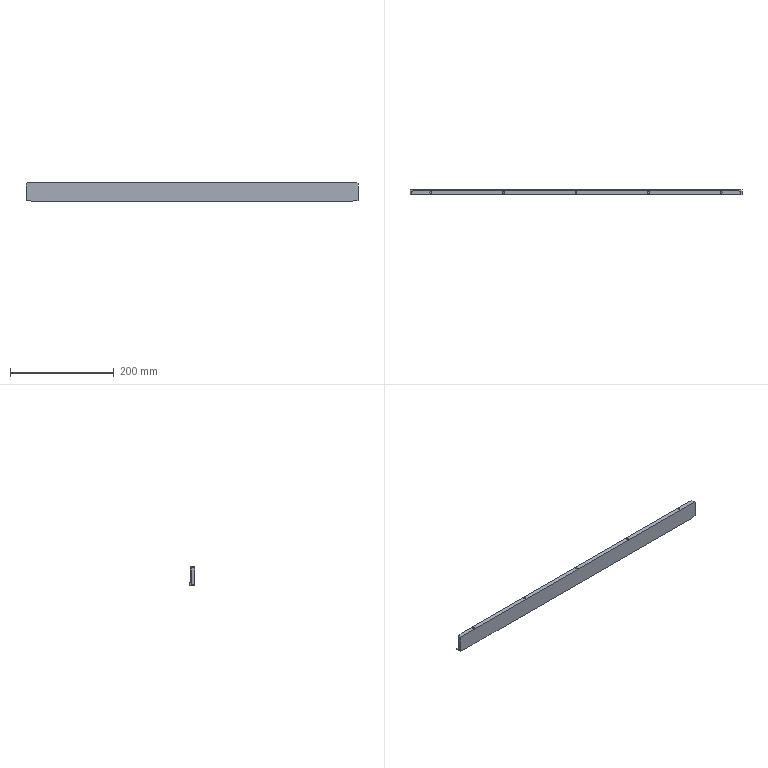Component | SolidWorks | XT-1-05-2-1 | 1 solid | 38 faces | box 640 x 10 x 35 mm | volume 184333 mm3 | plane 18 | cylinder 10 | cone 10 | commonest cylinder face diameters 3.3 x10
build123d program:
from build123d import *
from OCP.BRepFilletAPI import BRepFilletAPI_MakeChamfer

# Parameters (mm, degrees)
BOSS_EXTRUDE1_DEPTH   = 640
M4_TAPPED_HOLE1_D     = 3.3
M4_TAPPED_HOLE1_DEPTH = 10.1
M4_TAPPED_HOLE1_TIP   = 0.9914
CHAMFER1_SIZE         = 10
CHAMFER1_SIZE2        = 2
CHAMFER2_SIZE         = 1
CHAMFER2_SIZE2        = 10
CHAMFER3_SIZE         = 10
CHAMFER3_SIZE2        = 1
CHAMFER4_SIZE         = 2


with BuildPart() as part:
    # Sketch1 → Boss-Extrude1 (new body)
    with BuildSketch(Plane.XY):
        Polygon((0, 0), (0, -10), (35, -10), (35, -2), (5, -2), (5, 0), align=None)
    extrude(amount=BOSS_EXTRUDE1_DEPTH)

    # M4 Tapped Hole1
    with Locations(Plane(origin=(35, 0, 0), x_dir=(0, 0, -1), z_dir=(1, 0, 0))):
        with Locations((-600, -6), (-460, -6), (-320, -6), (-180, -6), (-40, -6)):
            Hole(M4_TAPPED_HOLE1_D / 2, depth=M4_TAPPED_HOLE1_DEPTH)
            with Locations((0, 0, -(M4_TAPPED_HOLE1_DEPTH + M4_TAPPED_HOLE1_TIP / 2))):  # 118° drill point
                Cone(0, M4_TAPPED_HOLE1_D / 2, M4_TAPPED_HOLE1_TIP, mode=Mode.SUBTRACT)

    # Chamfer1: one chamfer whose edges measure the first distance from different faces: ONE call of the kernel's chamfer builder (chamfer() names one face for all edges)
    chamfer1_edges_1 = [part.edges().sort_by_distance(p)[0] for p in [
        (20, -2, 640),
        (20, -2, 0),
    ]]
    chamfer1_side_1 = [part.faces().sort_by_distance(p)[0] for p in [
        (20, -2, 320),
    ]]
    chamfer1_edges_2 = [part.edges().sort_by_distance(p)[0] for p in [
        (5, -1, 640),
        (5, -1, 0),
    ]]
    chamfer1_side_2 = [part.faces().sort_by_distance(p)[0] for p in [
        (5, -1, 320),
    ]]
    chamfer1 = BRepFilletAPI_MakeChamfer(part.part.solid().wrapped)
    for e in chamfer1_edges_1:
        chamfer1.Add(CHAMFER1_SIZE, CHAMFER1_SIZE2, e.wrapped, chamfer1_side_1[0].wrapped)  # the first distance lies on this face
    for e in chamfer1_edges_2:
        chamfer1.Add(CHAMFER1_SIZE, CHAMFER1_SIZE2, e.wrapped, chamfer1_side_2[0].wrapped)  # the first distance lies on this face
    add(Compound.cast(chamfer1.Shape()), mode=Mode.REPLACE)

    # Chamfer2
    chamfer2_edges = [part.edges().sort_by_distance(p)[0] for p in [
        (1.5, 0, 0),
        (0, -5, 0),
    ]]
    chamfer2_side = [part.faces().sort_by_distance(p)[0] for p in [
        (16.635, -6.73, 0),
    ]]
    chamfer(chamfer2_edges, length=CHAMFER2_SIZE, length2=CHAMFER2_SIZE2, reference=chamfer2_side[0])

    # Chamfer3: one chamfer whose edges measure the first distance from different faces: ONE call of the kernel's chamfer builder (chamfer() names one face for all edges)
    chamfer3_edges_1 = [part.edges().sort_by_distance(p)[0] for p in [
        (1.5, 0, 640),
    ]]
    chamfer3_side_1 = [part.faces().sort_by_distance(p)[0] for p in [
        (2.494, 0, 324.007),
    ]]
    chamfer3_edges_2 = [part.edges().sort_by_distance(p)[0] for p in [
        (0, -5, 640),
    ]]
    chamfer3_side_2 = [part.faces().sort_by_distance(p)[0] for p in [
        (0, -5, 325),
    ]]
    chamfer3 = BRepFilletAPI_MakeChamfer(part.part.solid().wrapped)
    for e in chamfer3_edges_1:
        chamfer3.Add(CHAMFER3_SIZE, CHAMFER3_SIZE2, e.wrapped, chamfer3_side_1[0].wrapped)  # the first distance lies on this face
    for e in chamfer3_edges_2:
        chamfer3.Add(CHAMFER3_SIZE, CHAMFER3_SIZE2, e.wrapped, chamfer3_side_2[0].wrapped)  # the first distance lies on this face
    add(Compound.cast(chamfer3.Shape()), mode=Mode.REPLACE)

    # Chamfer4
    chamfer4_edges = [part.edges().sort_by_distance(p)[0] for p in [
        (35, -7, 640),
        (35, -7, 0),
    ]]
    chamfer(chamfer4_edges, length=CHAMFER4_SIZE)


solid = part.part

# Placed as in the assembly
solid = solid.moved(Location((909.283, 131.385, -42.5), (0, -90, 0)))
STEP:
#1=COLOUR_RGB('',0.7922,0.8196,0.9333);
#2=FILL_AREA_STYLE_COLOUR('',#1);
#3=FILL_AREA_STYLE('',(#2));
#4=SURFACE_STYLE_FILL_AREA(#3);
#5=SURFACE_SIDE_STYLE('',(#4));
#6=SURFACE_STYLE_USAGE(.BOTH.,#5);
#7=PRESENTATION_STYLE_ASSIGNMENT((#6));
#8=CARTESIAN_POINT('',(12.112,4.936,-0.6929));
#9=VERTEX_POINT('',#8);
#10=CARTESIAN_POINT('',(12.241,4.936,-0.6929));
#11=VERTEX_POINT('',#10);
#12=CARTESIAN_POINT('',(12.177,4.936,-0.6929));
#13=DIRECTION('',(0.,0.,1.));
#14=DIRECTION('',(1.,0.,0.));
#15=AXIS2_PLACEMENT_3D('',#12,#13,#14);
#16=CIRCLE('',#15,0.06496);
#17=EDGE_CURVE('',#9,#11,#16,.T.);
#18=ORIENTED_EDGE('',*,*,#17,.F.);
#19=CARTESIAN_POINT('',(12.112,4.936,-0.2953));
#20=VERTEX_POINT('',#19);
#21=CARTESIAN_POINT('',(12.112,4.936,-0.2953));
#22=DIRECTION('',(0.,0.,1.));
#23=VECTOR('',#22,39.37);
#24=LINE('',#21,#23);
#25=EDGE_CURVE('',#9,#20,#24,.T.);
#26=ORIENTED_EDGE('',*,*,#25,.T.);
#27=CARTESIAN_POINT('',(12.241,4.936,-0.2953));
#28=VERTEX_POINT('',#27);
#29=CARTESIAN_POINT('',(12.177,4.936,-0.2953));
#30=DIRECTION('',(0.,0.,1.));
#31=DIRECTION('',(1.,0.,0.));
#32=AXIS2_PLACEMENT_3D('',#29,#30,#31);
#33=CIRCLE('',#32,0.06496);
#34=EDGE_CURVE('',#20,#28,#33,.T.);
#35=ORIENTED_EDGE('',*,*,#34,.T.);
#36=CARTESIAN_POINT('',(12.241,4.936,-0.2953));
#37=DIRECTION('',(0.,0.,1.));
#38=VECTOR('',#37,39.37);
#39=LINE('',#36,#38);
#40=EDGE_CURVE('',#11,#28,#39,.T.);
#41=ORIENTED_EDGE('',*,*,#40,.F.);
#42=EDGE_LOOP('',(#18,#26,#35,#41));
#43=FACE_OUTER_BOUND('',#42,.T.);
#44=CARTESIAN_POINT('',(12.177,4.936,-0.2953));
#45=DIRECTION('',(0.,0.,1.));
#46=DIRECTION('',(1.,0.,0.));
#47=AXIS2_PLACEMENT_3D('',#44,#45,#46);
#48=CYLINDRICAL_SURFACE('',#47,0.06496);
#49=ADVANCED_FACE('',(#43),#48,.F.);
#50=CARTESIAN_POINT('',(12.177,4.936,-0.7319));
#51=VERTEX_POINT('',#50);
#52=CARTESIAN_POINT('',(12.241,4.936,-0.6929));
#53=DIRECTION('',(0.8572,0.,0.515));
#54=VECTOR('',#53,39.37);
#55=LINE('',#52,#54);
#56=EDGE_CURVE('',#51,#11,#55,.T.);
#57=ORIENTED_EDGE('',*,*,#56,.F.);
#58=CARTESIAN_POINT('',(12.112,4.936,-0.6929));
#59=DIRECTION('',(-0.8572,0.,0.515));
#60=VECTOR('',#59,39.37);
#61=LINE('',#58,#60);
#62=EDGE_CURVE('',#51,#9,#61,.T.);
#63=ORIENTED_EDGE('',*,*,#62,.T.);
#64=ORIENTED_EDGE('',*,*,#17,.T.);
#65=EDGE_LOOP('',(#57,#63,#64));
#66=FACE_OUTER_BOUND('',#65,.T.);
#67=CARTESIAN_POINT('',(12.177,4.936,-0.6929));
#68=DIRECTION('',(0.,0.,1.));
#69=DIRECTION('',(1.,0.,0.));
#70=AXIS2_PLACEMENT_3D('',#67,#68,#69);
#71=CONICAL_SURFACE('',#70,0.06496,1.03);
#72=ADVANCED_FACE('',(#66),#71,.F.);
#73=CARTESIAN_POINT('',(17.623,4.936,-0.6929));
#74=VERTEX_POINT('',#73);
#75=CARTESIAN_POINT('',(17.753,4.936,-0.6929));
#76=VERTEX_POINT('',#75);
#77=CARTESIAN_POINT('',(17.688,4.936,-0.6929));
#78=DIRECTION('',(0.,0.,1.));
#79=DIRECTION('',(1.,0.,0.));
#80=AXIS2_PLACEMENT_3D('',#77,#78,#79);
#81=CIRCLE('',#80,0.06496);
#82=EDGE_CURVE('',#74,#76,#81,.T.);
#83=ORIENTED_EDGE('',*,*,#82,.F.);
#84=CARTESIAN_POINT('',(17.623,4.936,-0.2953));
#85=VERTEX_POINT('',#84);
#86=CARTESIAN_POINT('',(17.623,4.936,-0.2953));
#87=DIRECTION('',(0.,0.,1.));
#88=VECTOR('',#87,39.37);
#89=LINE('',#86,#88);
#90=EDGE_CURVE('',#74,#85,#89,.T.);
#91=ORIENTED_EDGE('',*,*,#90,.T.);
#92=CARTESIAN_POINT('',(17.753,4.936,-0.2953));
#93=VERTEX_POINT('',#92);
#94=CARTESIAN_POINT('',(17.688,4.936,-0.2953));
#95=DIRECTION('',(0.,0.,1.));
#96=DIRECTION('',(1.,0.,0.));
#97=AXIS2_PLACEMENT_3D('',#94,#95,#96);
#98=CIRCLE('',#97,0.06496);
#99=EDGE_CURVE('',#85,#93,#98,.T.);
#100=ORIENTED_EDGE('',*,*,#99,.T.);
#101=CARTESIAN_POINT('',(17.753,4.936,-0.2953));
#102=DIRECTION('',(0.,0.,1.));
#103=VECTOR('',#102,39.37);
#104=LINE('',#101,#103);
#105=EDGE_CURVE('',#76,#93,#104,.T.);
#106=ORIENTED_EDGE('',*,*,#105,.F.);
#107=EDGE_LOOP('',(#83,#91,#100,#106));
#108=FACE_OUTER_BOUND('',#107,.T.);
#109=CARTESIAN_POINT('',(17.688,4.936,-0.2953));
#110=DIRECTION('',(0.,0.,1.));
#111=DIRECTION('',(1.,0.,0.));
#112=AXIS2_PLACEMENT_3D('',#109,#110,#111);
#113=CYLINDRICAL_SURFACE('',#112,0.06496);
#114=ADVANCED_FACE('',(#108),#113,.F.);
#115=CARTESIAN_POINT('',(17.688,4.936,-0.7319));
#116=VERTEX_POINT('',#115);
#117=CARTESIAN_POINT('',(17.753,4.936,-0.6929));
#118=DIRECTION('',(0.8572,0.,0.515));
#119=VECTOR('',#118,39.37);
#120=LINE('',#117,#119);
#121=EDGE_CURVE('',#116,#76,#120,.T.);
#122=ORIENTED_EDGE('',*,*,#121,.F.);
#123=CARTESIAN_POINT('',(17.623,4.936,-0.6929));
#124=DIRECTION('',(-0.8572,0.,0.515));
#125=VECTOR('',#124,39.37);
#126=LINE('',#123,#125);
#127=EDGE_CURVE('',#116,#74,#126,.T.);
#128=ORIENTED_EDGE('',*,*,#127,.T.);
#129=ORIENTED_EDGE('',*,*,#82,.T.);
#130=EDGE_LOOP('',(#122,#128,#129));
#131=FACE_OUTER_BOUND('',#130,.T.);
#132=CARTESIAN_POINT('',(17.688,4.936,-0.6929));
#133=DIRECTION('',(0.,0.,1.));
#134=DIRECTION('',(1.,0.,0.));
#135=AXIS2_PLACEMENT_3D('',#132,#133,#134);
#136=CONICAL_SURFACE('',#135,0.06496,1.03);
#137=ADVANCED_FACE('',(#131),#136,.F.);
#138=CARTESIAN_POINT('',(23.135,4.936,-0.6929));
#139=VERTEX_POINT('',#138);
#140=CARTESIAN_POINT('',(23.265,4.936,-0.6929));
#141=VERTEX_POINT('',#140);
#142=CARTESIAN_POINT('',(23.2,4.936,-0.6929));
#143=DIRECTION('',(0.,0.,1.));
#144=DIRECTION('',(1.,0.,0.));
#145=AXIS2_PLACEMENT_3D('',#142,#143,#144);
#146=CIRCLE('',#145,0.06496);
#147=EDGE_CURVE('',#139,#141,#146,.T.);
#148=ORIENTED_EDGE('',*,*,#147,.F.);
#149=CARTESIAN_POINT('',(23.135,4.936,-0.2953));
#150=VERTEX_POINT('',#149);
#151=CARTESIAN_POINT('',(23.135,4.936,-0.2953));
#152=DIRECTION('',(0.,0.,1.));
#153=VECTOR('',#152,39.37);
#154=LINE('',#151,#153);
#155=EDGE_CURVE('',#139,#150,#154,.T.);
#156=ORIENTED_EDGE('',*,*,#155,.T.);
#157=CARTESIAN_POINT('',(23.265,4.936,-0.2953));
#158=VERTEX_POINT('',#157);
#159=CARTESIAN_POINT('',(23.2,4.936,-0.2953));
#160=DIRECTION('',(0.,0.,1.));
#161=DIRECTION('',(1.,0.,0.));
#162=AXIS2_PLACEMENT_3D('',#159,#160,#161);
#163=CIRCLE('',#162,0.06496);
#164=EDGE_CURVE('',#150,#158,#163,.T.);
#165=ORIENTED_EDGE('',*,*,#164,.T.);
#166=CARTESIAN_POINT('',(23.265,4.936,-0.2953));
#167=DIRECTION('',(0.,0.,1.));
#168=VECTOR('',#167,39.37);
#169=LINE('',#166,#168);
#170=EDGE_CURVE('',#141,#158,#169,.T.);
#171=ORIENTED_EDGE('',*,*,#170,.F.);
#172=EDGE_LOOP('',(#148,#156,#165,#171));
#173=FACE_OUTER_BOUND('',#172,.T.);
#174=CARTESIAN_POINT('',(23.2,4.936,-0.2953));
#175=DIRECTION('',(0.,0.,1.));
#176=DIRECTION('',(1.,0.,0.));
#177=AXIS2_PLACEMENT_3D('',#174,#175,#176);
#178=CYLINDRICAL_SURFACE('',#177,0.06496);
#179=ADVANCED_FACE('',(#173),#178,.F.);
#180=CARTESIAN_POINT('',(23.2,4.936,-0.7319));
#181=VERTEX_POINT('',#180);
#182=CARTESIAN_POINT('',(23.265,4.936,-0.6929));
#183=DIRECTION('',(0.8572,0.,0.515));
#184=VECTOR('',#183,39.37);
#185=LINE('',#182,#184);
#186=EDGE_CURVE('',#181,#141,#185,.T.);
#187=ORIENTED_EDGE('',*,*,#186,.F.);
#188=CARTESIAN_POINT('',(23.135,4.936,-0.6929));
#189=DIRECTION('',(-0.8572,0.,0.515));
#190=VECTOR('',#189,39.37);
#191=LINE('',#188,#190);
#192=EDGE_CURVE('',#181,#139,#191,.T.);
#193=ORIENTED_EDGE('',*,*,#192,.T.);
#194=ORIENTED_EDGE('',*,*,#147,.T.);
#195=EDGE_LOOP('',(#187,#193,#194));
#196=FACE_OUTER_BOUND('',#195,.T.);
#197=CARTESIAN_POINT('',(23.2,4.936,-0.6929));
#198=DIRECTION('',(0.,0.,1.));
#199=DIRECTION('',(1.,0.,0.));
#200=AXIS2_PLACEMENT_3D('',#197,#198,#199);
#201=CONICAL_SURFACE('',#200,0.06496,1.03);
#202=ADVANCED_FACE('',(#196),#201,.F.);
#203=CARTESIAN_POINT('',(28.647,4.936,-0.6929));
#204=VERTEX_POINT('',#203);
#205=CARTESIAN_POINT('',(28.777,4.936,-0.6929));
#206=VERTEX_POINT('',#205);
#207=CARTESIAN_POINT('',(28.712,4.936,-0.6929));
#208=DIRECTION('',(0.,0.,1.));
#209=DIRECTION('',(1.,0.,0.));
#210=AXIS2_PLACEMENT_3D('',#207,#208,#209);
#211=CIRCLE('',#210,0.06496);
#212=EDGE_CURVE('',#204,#206,#211,.T.);
#213=ORIENTED_EDGE('',*,*,#212,.F.);
#214=CARTESIAN_POINT('',(28.647,4.936,-0.2953));
#215=VERTEX_POINT('',#214);
#216=CARTESIAN_POINT('',(28.647,4.936,-0.2953));
#217=DIRECTION('',(0.,0.,1.));
#218=VECTOR('',#217,39.37);
#219=LINE('',#216,#218);
#220=EDGE_CURVE('',#204,#215,#219,.T.);
#221=ORIENTED_EDGE('',*,*,#220,.T.);
#222=CARTESIAN_POINT('',(28.777,4.936,-0.2953));
#223=VERTEX_POINT('',#222);
#224=CARTESIAN_POINT('',(28.712,4.936,-0.2953));
#225=DIRECTION('',(0.,0.,1.));
#226=DIRECTION('',(1.,0.,0.));
#227=AXIS2_PLACEMENT_3D('',#224,#225,#226);
#228=CIRCLE('',#227,0.06496);
#229=EDGE_CURVE('',#215,#223,#228,.T.);
#230=ORIENTED_EDGE('',*,*,#229,.T.);
#231=CARTESIAN_POINT('',(28.777,4.936,-0.2953));
#232=DIRECTION('',(0.,0.,1.));
#233=VECTOR('',#232,39.37);
#234=LINE('',#231,#233);
#235=EDGE_CURVE('',#206,#223,#234,.T.);
#236=ORIENTED_EDGE('',*,*,#235,.F.);
#237=EDGE_LOOP('',(#213,#221,#230,#236));
#238=FACE_OUTER_BOUND('',#237,.T.);
#239=CARTESIAN_POINT('',(28.712,4.936,-0.2953));
#240=DIRECTION('',(0.,0.,1.));
#241=DIRECTION('',(1.,0.,0.));
#242=AXIS2_PLACEMENT_3D('',#239,#240,#241);
#243=CYLINDRICAL_SURFACE('',#242,0.06496);
#244=ADVANCED_FACE('',(#238),#243,.F.);
#245=CARTESIAN_POINT('',(28.712,4.936,-0.7319));
#246=VERTEX_POINT('',#245);
#247=CARTESIAN_POINT('',(28.777,4.936,-0.6929));
#248=DIRECTION('',(0.8572,0.,0.515));
#249=VECTOR('',#248,39.37);
#250=LINE('',#247,#249);
#251=EDGE_CURVE('',#246,#206,#250,.T.);
#252=ORIENTED_EDGE('',*,*,#251,.F.);
#253=CARTESIAN_POINT('',(28.647,4.936,-0.6929));
#254=DIRECTION('',(-0.8572,0.,0.515));
#255=VECTOR('',#254,39.37);
#256=LINE('',#253,#255);
#257=EDGE_CURVE('',#246,#204,#256,.T.);
#258=ORIENTED_EDGE('',*,*,#257,.T.);
#259=ORIENTED_EDGE('',*,*,#212,.T.);
#260=EDGE_LOOP('',(#252,#258,#259));
#261=FACE_OUTER_BOUND('',#260,.T.);
#262=CARTESIAN_POINT('',(28.712,4.936,-0.6929));
#263=DIRECTION('',(0.,0.,1.));
#264=DIRECTION('',(1.,0.,0.));
#265=AXIS2_PLACEMENT_3D('',#262,#263,#264);
#266=CONICAL_SURFACE('',#265,0.06496,1.03);
#267=ADVANCED_FACE('',(#261),#266,.F.);
#268=CARTESIAN_POINT('',(34.159,4.936,-0.6929));
#269=VERTEX_POINT('',#268);
#270=CARTESIAN_POINT('',(34.289,4.936,-0.6929));
#271=VERTEX_POINT('',#270);
#272=CARTESIAN_POINT('',(34.224,4.936,-0.6929));
#273=DIRECTION('',(0.,0.,1.));
#274=DIRECTION('',(1.,0.,0.));
#275=AXIS2_PLACEMENT_3D('',#272,#273,#274);
#276=CIRCLE('',#275,0.06496);
#277=EDGE_CURVE('',#269,#271,#276,.T.);
#278=ORIENTED_EDGE('',*,*,#277,.F.);
#279=CARTESIAN_POINT('',(34.159,4.936,-0.2953));
#280=VERTEX_POINT('',#279);
#281=CARTESIAN_POINT('',(34.159,4.936,-0.2953));
#282=DIRECTION('',(0.,0.,1.));
#283=VECTOR('',#282,39.37);
#284=LINE('',#281,#283);
#285=EDGE_CURVE('',#269,#280,#284,.T.);
#286=ORIENTED_EDGE('',*,*,#285,.T.);
#287=CARTESIAN_POINT('',(34.289,4.936,-0.2953));
#288=VERTEX_POINT('',#287);
#289=CARTESIAN_POINT('',(34.224,4.936,-0.2953));
#290=DIRECTION('',(0.,0.,1.));
#291=DIRECTION('',(1.,0.,0.));
#292=AXIS2_PLACEMENT_3D('',#289,#290,#291);
#293=CIRCLE('',#292,0.06496);
#294=EDGE_CURVE('',#280,#288,#293,.T.);
#295=ORIENTED_EDGE('',*,*,#294,.T.);
#296=CARTESIAN_POINT('',(34.289,4.936,-0.2953));
#297=DIRECTION('',(0.,0.,1.));
#298=VECTOR('',#297,39.37);
#299=LINE('',#296,#298);
#300=EDGE_CURVE('',#271,#288,#299,.T.);
#301=ORIENTED_EDGE('',*,*,#300,.F.);
#302=EDGE_LOOP('',(#278,#286,#295,#301));
#303=FACE_OUTER_BOUND('',#302,.T.);
#304=CARTESIAN_POINT('',(34.224,4.936,-0.2953));
#305=DIRECTION('',(0.,0.,1.));
#306=DIRECTION('',(1.,0.,0.));
#307=AXIS2_PLACEMENT_3D('',#304,#305,#306);
#308=CYLINDRICAL_SURFACE('',#307,0.06496);
#309=ADVANCED_FACE('',(#303),#308,.F.);
#310=CARTESIAN_POINT('',(34.224,4.936,-0.7319));
#311=VERTEX_POINT('',#310);
#312=CARTESIAN_POINT('',(34.289,4.936,-0.6929));
#313=DIRECTION('',(0.8572,0.,0.515));
#314=VECTOR('',#313,39.37);
#315=LINE('',#312,#314);
#316=EDGE_CURVE('',#311,#271,#315,.T.);
#317=ORIENTED_EDGE('',*,*,#316,.F.);
#318=CARTESIAN_POINT('',(34.159,4.936,-0.6929));
#319=DIRECTION('',(-0.8572,0.,0.515));
#320=VECTOR('',#319,39.37);
#321=LINE('',#318,#320);
#322=EDGE_CURVE('',#311,#269,#321,.T.);
#323=ORIENTED_EDGE('',*,*,#322,.T.);
#324=ORIENTED_EDGE('',*,*,#277,.T.);
#325=EDGE_LOOP('',(#317,#323,#324));
#326=FACE_OUTER_BOUND('',#325,.T.);
#327=CARTESIAN_POINT('',(34.224,4.936,-0.6929));
#328=DIRECTION('',(0.,0.,1.));
#329=DIRECTION('',(1.,0.,0.));
#330=AXIS2_PLACEMENT_3D('',#327,#328,#329);
#331=CONICAL_SURFACE('',#330,0.06496,1.03);
#332=ADVANCED_FACE('',(#326),#331,.F.);
#333=CARTESIAN_POINT('',(10.995,5.173,-1.673));
#334=VERTEX_POINT('',#333);
#335=CARTESIAN_POINT('',(35.405,5.173,-1.673));
#336=VERTEX_POINT('',#335);
#337=CARTESIAN_POINT('',(10.602,5.173,-1.673));
#338=DIRECTION('',(1.,0.,0.));
#339=VECTOR('',#338,39.37);
#340=LINE('',#337,#339);
#341=EDGE_CURVE('',#334,#336,#340,.T.);
#342=ORIENTED_EDGE('',*,*,#341,.F.);
#343=CARTESIAN_POINT('',(10.995,5.173,-1.476));
#344=VERTEX_POINT('',#343);
#345=CARTESIAN_POINT('',(10.995,5.173,-1.555));
#346=DIRECTION('',(0.,0.,1.));
#347=VECTOR('',#346,39.37);
#348=LINE('',#345,#347);
#349=EDGE_CURVE('',#334,#344,#348,.T.);
#350=ORIENTED_EDGE('',*,*,#349,.T.);
#351=CARTESIAN_POINT('',(35.405,5.173,-1.476));
#352=VERTEX_POINT('',#351);
#353=CARTESIAN_POINT('',(10.602,5.173,-1.476));
#354=DIRECTION('',(1.,0.,0.));
#355=VECTOR('',#354,39.37);
#356=LINE('',#353,#355);
#357=EDGE_CURVE('',#344,#352,#356,.T.);
#358=ORIENTED_EDGE('',*,*,#357,.T.);
#359=CARTESIAN_POINT('',(35.405,5.173,-1.476));
#360=DIRECTION('',(0.,-0.,-1.));
#361=VECTOR('',#360,39.37);
#362=LINE('',#359,#361);
#363=EDGE_CURVE('',#352,#336,#362,.T.);
#364=ORIENTED_EDGE('',*,*,#363,.T.);
#365=EDGE_LOOP('',(#342,#350,#358,#364));
#366=FACE_OUTER_BOUND('',#365,.T.);
#367=CARTESIAN_POINT('',(10.602,5.173,-1.476));
#368=DIRECTION('',(0.,-1.,0.));
#369=DIRECTION('',(0.,0.,1.));
#370=AXIS2_PLACEMENT_3D('',#367,#368,#369);
#371=PLANE('',#370);
#372=ADVANCED_FACE('',(#366),#371,.F.);
#373=CARTESIAN_POINT('',(10.995,4.779,-1.673));
#374=VERTEX_POINT('',#373);
#375=CARTESIAN_POINT('',(35.405,4.779,-1.673));
#376=VERTEX_POINT('',#375);
#377=CARTESIAN_POINT('',(10.602,4.779,-1.673));
#378=DIRECTION('',(1.,0.,0.));
#379=VECTOR('',#378,39.37);
#380=LINE('',#377,#379);
#381=EDGE_CURVE('',#374,#376,#380,.T.);
#382=ORIENTED_EDGE('',*,*,#381,.F.);
#383=CARTESIAN_POINT('',(10.995,5.173,-1.673));
#384=DIRECTION('',(0.,1.,-0.));
#385=VECTOR('',#384,39.37);
#386=LINE('',#383,#385);
#387=EDGE_CURVE('',#374,#334,#386,.T.);
#388=ORIENTED_EDGE('',*,*,#387,.T.);
#389=ORIENTED_EDGE('',*,*,#341,.T.);
#390=CARTESIAN_POINT('',(35.405,5.173,-1.673));
#391=DIRECTION('',(0.,-1.,0.));
#392=VECTOR('',#391,39.37);
#393=LINE('',#390,#392);
#394=EDGE_CURVE('',#336,#376,#393,.T.);
#395=ORIENTED_EDGE('',*,*,#394,.T.);
#396=EDGE_LOOP('',(#382,#388,#389,#395));
#397=FACE_OUTER_BOUND('',#396,.T.);
#398=CARTESIAN_POINT('',(10.602,5.173,-1.673));
#399=DIRECTION('',(0.,0.,1.));
#400=DIRECTION('',(0.,1.,-0.));
#401=AXIS2_PLACEMENT_3D('',#398,#399,#400);
#402=PLANE('',#401);
#403=ADVANCED_FACE('',(#397),#402,.F.);
#404=CARTESIAN_POINT('',(35.799,4.779,-1.634));
#405=VERTEX_POINT('',#404);
#406=CARTESIAN_POINT('',(35.799,4.779,-0.374));
#407=VERTEX_POINT('',#406);
#408=CARTESIAN_POINT('',(35.799,4.779,-1.673));
#409=DIRECTION('',(0.,0.,1.));
#410=VECTOR('',#409,39.37);
#411=LINE('',#408,#410);
#412=EDGE_CURVE('',#405,#407,#411,.T.);
#413=ORIENTED_EDGE('',*,*,#412,.T.);
#414=CARTESIAN_POINT('',(35.72,4.779,-0.2953));
#415=VERTEX_POINT('',#414);
#416=CARTESIAN_POINT('',(35.72,4.779,-0.2953));
#417=DIRECTION('',(-0.7071,0.,0.7071));
#418=VECTOR('',#417,39.37);
#419=LINE('',#416,#418);
#420=EDGE_CURVE('',#407,#415,#419,.T.);
#421=ORIENTED_EDGE('',*,*,#420,.T.);
#422=CARTESIAN_POINT('',(10.68,4.779,-0.2953));
#423=VERTEX_POINT('',#422);
#424=CARTESIAN_POINT('',(10.602,4.779,-0.2953));
#425=DIRECTION('',(1.,0.,0.));
#426=VECTOR('',#425,39.37);
#427=LINE('',#424,#426);
#428=EDGE_CURVE('',#423,#415,#427,.T.);
#429=ORIENTED_EDGE('',*,*,#428,.F.);
#430=CARTESIAN_POINT('',(10.602,4.779,-0.374));
#431=VERTEX_POINT('',#430);
#432=CARTESIAN_POINT('',(10.602,4.779,-0.374));
#433=DIRECTION('',(-0.7071,-0.,-0.7071));
#434=VECTOR('',#433,39.37);
#435=LINE('',#432,#434);
#436=EDGE_CURVE('',#423,#431,#435,.T.);
#437=ORIENTED_EDGE('',*,*,#436,.T.);
#438=CARTESIAN_POINT('',(10.602,4.779,-1.634));
#439=VERTEX_POINT('',#438);
#440=CARTESIAN_POINT('',(10.602,4.779,-1.673));
#441=DIRECTION('',(0.,0.,1.));
#442=VECTOR('',#441,39.37);
#443=LINE('',#440,#442);
#444=EDGE_CURVE('',#439,#431,#443,.T.);
#445=ORIENTED_EDGE('',*,*,#444,.F.);
#446=CARTESIAN_POINT('',(10.602,4.779,-1.634));
#447=DIRECTION('',(0.995,-0.,-0.0995));
#448=VECTOR('',#447,39.37);
#449=LINE('',#446,#448);
#450=EDGE_CURVE('',#439,#374,#449,.T.);
#451=ORIENTED_EDGE('',*,*,#450,.T.);
#452=ORIENTED_EDGE('',*,*,#381,.T.);
#453=CARTESIAN_POINT('',(35.405,4.779,-1.673));
#454=DIRECTION('',(0.995,0.,0.0995));
#455=VECTOR('',#454,39.37);
#456=LINE('',#453,#455);
#457=EDGE_CURVE('',#376,#405,#456,.T.);
#458=ORIENTED_EDGE('',*,*,#457,.T.);
#459=EDGE_LOOP('',(#413,#421,#429,#437,#445,#451,#452,#458));
#460=FACE_OUTER_BOUND('',#459,.T.);
#461=CARTESIAN_POINT('',(10.602,4.779,-1.673));
#462=DIRECTION('',(0.,1.,-0.));
#463=DIRECTION('',(0.,-0.,-1.));
#464=AXIS2_PLACEMENT_3D('',#461,#462,#463);
#465=PLANE('',#464);
#466=ADVANCED_FACE('',(#460),#465,.F.);
#467=CARTESIAN_POINT('',(12.177,4.936,-0.2953));
#468=DIRECTION('',(0.,0.,1.));
#469=DIRECTION('',(1.,0.,0.));
#470=AXIS2_PLACEMENT_3D('',#467,#468,#469);
#471=CIRCLE('',#470,0.06496);
#472=EDGE_CURVE('',#28,#20,#471,.T.);
#473=ORIENTED_EDGE('',*,*,#472,.F.);
#474=ORIENTED_EDGE('',*,*,#34,.F.);
#475=EDGE_LOOP('',(#473,#474));
#476=FACE_BOUND('',#475,.T.);
#477=CARTESIAN_POINT('',(17.688,4.936,-0.2953));
#478=DIRECTION('',(0.,0.,1.));
#479=DIRECTION('',(1.,0.,0.));
#480=AXIS2_PLACEMENT_3D('',#477,#478,#479);
#481=CIRCLE('',#480,0.06496);
#482=EDGE_CURVE('',#93,#85,#481,.T.);
#483=ORIENTED_EDGE('',*,*,#482,.F.);
#484=ORIENTED_EDGE('',*,*,#99,.F.);
#485=EDGE_LOOP('',(#483,#484));
#486=FACE_BOUND('',#485,.T.);
#487=CARTESIAN_POINT('',(23.2,4.936,-0.2953));
#488=DIRECTION('',(0.,0.,1.));
#489=DIRECTION('',(1.,0.,0.));
#490=AXIS2_PLACEMENT_3D('',#487,#488,#489);
#491=CIRCLE('',#490,0.06496);
#492=EDGE_CURVE('',#158,#150,#491,.T.);
#493=ORIENTED_EDGE('',*,*,#492,.F.);
#494=ORIENTED_EDGE('',*,*,#164,.F.);
#495=EDGE_LOOP('',(#493,#494));
#496=FACE_BOUND('',#495,.T.);
#497=CARTESIAN_POINT('',(28.712,4.936,-0.2953));
#498=DIRECTION('',(0.,0.,1.));
#499=DIRECTION('',(1.,0.,0.));
#500=AXIS2_PLACEMENT_3D('',#497,#498,#499);
#501=CIRCLE('',#500,0.06496);
#502=EDGE_CURVE('',#223,#215,#501,.T.);
#503=ORIENTED_EDGE('',*,*,#502,.F.);
#504=ORIENTED_EDGE('',*,*,#229,.F.);
#505=EDGE_LOOP('',(#503,#504));
#506=FACE_BOUND('',#505,.T.);
#507=CARTESIAN_POINT('',(34.224,4.936,-0.2953));
#508=DIRECTION('',(0.,0.,1.));
#509=DIRECTION('',(1.,0.,0.));
#510=AXIS2_PLACEMENT_3D('',#507,#508,#509);
#511=CIRCLE('',#510,0.06496);
#512=EDGE_CURVE('',#288,#280,#511,.T.);
#513=ORIENTED_EDGE('',*,*,#512,.F.);
#514=ORIENTED_EDGE('',*,*,#294,.F.);
#515=EDGE_LOOP('',(#513,#514));
#516=FACE_BOUND('',#515,.T.);
#517=ORIENTED_EDGE('',*,*,#428,.T.);
#518=CARTESIAN_POINT('',(35.72,5.031,-0.2953));
#519=VERTEX_POINT('',#518);
#520=CARTESIAN_POINT('',(35.72,4.779,-0.2953));
#521=DIRECTION('',(0.,1.,0.));
#522=VECTOR('',#521,39.37);
#523=LINE('',#520,#522);
#524=EDGE_CURVE('',#415,#519,#523,.T.);
#525=ORIENTED_EDGE('',*,*,#524,.T.);
#526=CARTESIAN_POINT('',(35.405,5.094,-0.2953));
#527=VERTEX_POINT('',#526);
#528=CARTESIAN_POINT('',(35.405,5.094,-0.2953));
#529=DIRECTION('',(-0.9806,0.1961,0.));
#530=VECTOR('',#529,39.37);
#531=LINE('',#528,#530);
#532=EDGE_CURVE('',#519,#527,#531,.T.);
#533=ORIENTED_EDGE('',*,*,#532,.T.);
#534=CARTESIAN_POINT('',(10.995,5.094,-0.2953));
#535=VERTEX_POINT('',#534);
#536=CARTESIAN_POINT('',(10.602,5.094,-0.2953));
#537=DIRECTION('',(1.,0.,0.));
#538=VECTOR('',#537,39.37);
#539=LINE('',#536,#538);
#540=EDGE_CURVE('',#535,#527,#539,.T.);
#541=ORIENTED_EDGE('',*,*,#540,.F.);
#542=CARTESIAN_POINT('',(10.68,5.031,-0.2953));
#543=VERTEX_POINT('',#542);
#544=CARTESIAN_POINT('',(10.602,5.015,-0.2953));
#545=DIRECTION('',(-0.9806,-0.1961,0.));
#546=VECTOR('',#545,39.37);
#547=LINE('',#544,#546);
#548=EDGE_CURVE('',#535,#543,#547,.T.);
#549=ORIENTED_EDGE('',*,*,#548,.T.);
#550=CARTESIAN_POINT('',(10.68,4.779,-0.2953));
#551=DIRECTION('',(0.,-1.,0.));
#552=VECTOR('',#551,39.37);
#553=LINE('',#550,#552);
#554=EDGE_CURVE('',#543,#423,#553,.T.);
#555=ORIENTED_EDGE('',*,*,#554,.T.);
#556=EDGE_LOOP('',(#517,#525,#533,#541,#549,#555));
#557=FACE_OUTER_BOUND('',#556,.T.);
#558=CARTESIAN_POINT('',(10.602,4.779,-0.2953));
#559=DIRECTION('',(0.,0.,-1.));
#560=DIRECTION('',(-1.,0.,0.));
#561=AXIS2_PLACEMENT_3D('',#558,#559,#560);
#562=PLANE('',#561);
#563=ADVANCED_FACE('',(#476,#486,#496,#506,#516,#557),#562,.F.);
#564=ORIENTED_EDGE('',*,*,#540,.T.);
#565=CARTESIAN_POINT('',(35.405,5.094,-1.476));
#566=VERTEX_POINT('',#565);
#567=CARTESIAN_POINT('',(35.405,5.094,-0.2953));
#568=DIRECTION('',(0.,-0.,-1.));
#569=VECTOR('',#568,39.37);
#570=LINE('',#567,#569);
#571=EDGE_CURVE('',#527,#566,#570,.T.);
#572=ORIENTED_EDGE('',*,*,#571,.T.);
#573=CARTESIAN_POINT('',(10.995,5.094,-1.476));
#574=VERTEX_POINT('',#573);
#575=CARTESIAN_POINT('',(10.602,5.094,-1.476));
#576=DIRECTION('',(1.,0.,0.));
#577=VECTOR('',#576,39.37);
#578=LINE('',#575,#577);
#579=EDGE_CURVE('',#574,#566,#578,.T.);
#580=ORIENTED_EDGE('',*,*,#579,.F.);
#581=CARTESIAN_POINT('',(10.995,5.094,-0.2953));
#582=DIRECTION('',(0.,0.,1.));
#583=VECTOR('',#582,39.37);
#584=LINE('',#581,#583);
#585=EDGE_CURVE('',#574,#535,#584,.T.);
#586=ORIENTED_EDGE('',*,*,#585,.T.);
#587=EDGE_LOOP('',(#564,#572,#580,#586));
#588=FACE_OUTER_BOUND('',#587,.T.);
#589=CARTESIAN_POINT('',(10.602,5.094,-0.2953));
#590=DIRECTION('',(0.,-1.,0.));
#591=DIRECTION('',(0.,0.,1.));
#592=AXIS2_PLACEMENT_3D('',#589,#590,#591);
#593=PLANE('',#592);
#594=ADVANCED_FACE('',(#588),#593,.F.);
#595=ORIENTED_EDGE('',*,*,#579,.T.);
#596=CARTESIAN_POINT('',(35.405,5.094,-1.476));
#597=DIRECTION('',(0.,1.,0.));
#598=VECTOR('',#597,39.37);
#599=LINE('',#596,#598);
#600=EDGE_CURVE('',#566,#352,#599,.T.);
#601=ORIENTED_EDGE('',*,*,#600,.T.);
#602=ORIENTED_EDGE('',*,*,#357,.F.);
#603=CARTESIAN_POINT('',(10.995,5.094,-1.476));
#604=DIRECTION('',(0.,-1.,0.));
#605=VECTOR('',#604,39.37);
#606=LINE('',#603,#605);
#607=EDGE_CURVE('',#344,#574,#606,.T.);
#608=ORIENTED_EDGE('',*,*,#607,.T.);
#609=EDGE_LOOP('',(#595,#601,#602,#608));
#610=FACE_OUTER_BOUND('',#609,.T.);
#611=CARTESIAN_POINT('',(10.602,5.094,-1.476));
#612=DIRECTION('',(0.,0.,-1.));
#613=DIRECTION('',(-1.,0.,0.));
#614=AXIS2_PLACEMENT_3D('',#611,#612,#613);
#615=PLANE('',#614);
#616=ADVANCED_FACE('',(#610),#615,.F.);
#617=ORIENTED_EDGE('',*,*,#444,.T.);
#618=CARTESIAN_POINT('',(10.602,5.015,-0.374));
#619=VERTEX_POINT('',#618);
#620=CARTESIAN_POINT('',(10.602,5.015,-0.374));
#621=DIRECTION('',(0.,1.,0.));
#622=VECTOR('',#621,39.37);
#623=LINE('',#620,#622);
#624=EDGE_CURVE('',#431,#619,#623,.T.);
#625=ORIENTED_EDGE('',*,*,#624,.T.);
#626=CARTESIAN_POINT('',(10.602,5.015,-1.555));
#627=VERTEX_POINT('',#626);
#628=CARTESIAN_POINT('',(10.602,5.015,-1.476));
#629=DIRECTION('',(0.,-0.,-1.));
#630=VECTOR('',#629,39.37);
#631=LINE('',#628,#630);
#632=EDGE_CURVE('',#619,#627,#631,.T.);
#633=ORIENTED_EDGE('',*,*,#632,.T.);
#634=CARTESIAN_POINT('',(10.602,5.133,-1.555));
#635=VERTEX_POINT('',#634);
#636=CARTESIAN_POINT('',(10.602,5.173,-1.555));
#637=DIRECTION('',(0.,1.,0.));
#638=VECTOR('',#637,39.37);
#639=LINE('',#636,#638);
#640=EDGE_CURVE('',#627,#635,#639,.T.);
#641=ORIENTED_EDGE('',*,*,#640,.T.);
#642=CARTESIAN_POINT('',(10.602,5.133,-1.634));
#643=VERTEX_POINT('',#642);
#644=CARTESIAN_POINT('',(10.602,5.133,-1.673));
#645=DIRECTION('',(0.,-0.,-1.));
#646=VECTOR('',#645,39.37);
#647=LINE('',#644,#646);
#648=EDGE_CURVE('',#635,#643,#647,.T.);
#649=ORIENTED_EDGE('',*,*,#648,.T.);
#650=CARTESIAN_POINT('',(10.602,4.779,-1.634));
#651=DIRECTION('',(0.,-1.,0.));
#652=VECTOR('',#651,39.37);
#653=LINE('',#650,#652);
#654=EDGE_CURVE('',#643,#439,#653,.T.);
#655=ORIENTED_EDGE('',*,*,#654,.T.);
#656=EDGE_LOOP('',(#617,#625,#633,#641,#649,#655));
#657=FACE_OUTER_BOUND('',#656,.T.);
#658=CARTESIAN_POINT('',(10.602,5.173,-1.673));
#659=DIRECTION('',(-1.,0.,0.));
#660=DIRECTION('',(0.,0.,1.));
#661=AXIS2_PLACEMENT_3D('',#658,#659,#660);
#662=PLANE('',#661);
#663=ADVANCED_FACE('',(#657),#662,.T.);
#664=CARTESIAN_POINT('',(35.799,5.015,-1.555));
#665=VERTEX_POINT('',#664);
#666=CARTESIAN_POINT('',(35.799,5.015,-0.374));
#667=VERTEX_POINT('',#666);
#668=CARTESIAN_POINT('',(35.799,5.015,-1.673));
#669=DIRECTION('',(0.,0.,1.));
#670=VECTOR('',#669,39.37);
#671=LINE('',#668,#670);
#672=EDGE_CURVE('',#665,#667,#671,.T.);
#673=ORIENTED_EDGE('',*,*,#672,.T.);
#674=CARTESIAN_POINT('',(35.799,5.173,-0.374));
#675=DIRECTION('',(0.,-1.,0.));
#676=VECTOR('',#675,39.37);
#677=LINE('',#674,#676);
#678=EDGE_CURVE('',#667,#407,#677,.T.);
#679=ORIENTED_EDGE('',*,*,#678,.T.);
#680=ORIENTED_EDGE('',*,*,#412,.F.);
#681=CARTESIAN_POINT('',(35.799,5.133,-1.634));
#682=VERTEX_POINT('',#681);
#683=CARTESIAN_POINT('',(35.799,5.173,-1.634));
#684=DIRECTION('',(0.,1.,-0.));
#685=VECTOR('',#684,39.37);
#686=LINE('',#683,#685);
#687=EDGE_CURVE('',#405,#682,#686,.T.);
#688=ORIENTED_EDGE('',*,*,#687,.T.);
#689=CARTESIAN_POINT('',(35.799,5.133,-1.555));
#690=VERTEX_POINT('',#689);
#691=CARTESIAN_POINT('',(35.799,5.133,-1.673));
#692=DIRECTION('',(0.,0.,1.));
#693=VECTOR('',#692,39.37);
#694=LINE('',#691,#693);
#695=EDGE_CURVE('',#682,#690,#694,.T.);
#696=ORIENTED_EDGE('',*,*,#695,.T.);
#697=CARTESIAN_POINT('',(35.799,5.173,-1.555));
#698=DIRECTION('',(0.,-1.,0.));
#699=VECTOR('',#698,39.37);
#700=LINE('',#697,#699);
#701=EDGE_CURVE('',#690,#665,#700,.T.);
#702=ORIENTED_EDGE('',*,*,#701,.T.);
#703=EDGE_LOOP('',(#673,#679,#680,#688,#696,#702));
#704=FACE_OUTER_BOUND('',#703,.T.);
#705=CARTESIAN_POINT('',(35.799,5.173,-1.673));
#706=DIRECTION('',(-1.,0.,0.));
#707=DIRECTION('',(0.,0.,1.));
#708=AXIS2_PLACEMENT_3D('',#705,#706,#707);
#709=PLANE('',#708);
#710=ADVANCED_FACE('',(#704),#709,.F.);
#711=ORIENTED_EDGE('',*,*,#322,.F.);
#712=ORIENTED_EDGE('',*,*,#316,.T.);
#713=CARTESIAN_POINT('',(34.224,4.936,-0.6929));
#714=DIRECTION('',(0.,0.,1.));
#715=DIRECTION('',(1.,0.,0.));
#716=AXIS2_PLACEMENT_3D('',#713,#714,#715);
#717=CIRCLE('',#716,0.06496);
#718=EDGE_CURVE('',#271,#269,#717,.T.);
#719=ORIENTED_EDGE('',*,*,#718,.T.);
#720=EDGE_LOOP('',(#711,#712,#719));
#721=FACE_OUTER_BOUND('',#720,.T.);
#722=CARTESIAN_POINT('',(34.224,4.936,-0.6929));
#723=DIRECTION('',(0.,0.,1.));
#724=DIRECTION('',(1.,0.,0.));
#725=AXIS2_PLACEMENT_3D('',#722,#723,#724);
#726=CONICAL_SURFACE('',#725,0.06496,1.03);
#727=ADVANCED_FACE('',(#721),#726,.F.);
#728=ORIENTED_EDGE('',*,*,#285,.F.);
#729=ORIENTED_EDGE('',*,*,#718,.F.);
#730=ORIENTED_EDGE('',*,*,#300,.T.);
#731=ORIENTED_EDGE('',*,*,#512,.T.);
#732=EDGE_LOOP('',(#728,#729,#730,#731));
#733=FACE_OUTER_BOUND('',#732,.T.);
#734=CARTESIAN_POINT('',(34.224,4.936,-0.2953));
#735=DIRECTION('',(0.,0.,1.));
#736=DIRECTION('',(1.,0.,0.));
#737=AXIS2_PLACEMENT_3D('',#734,#735,#736);
#738=CYLINDRICAL_SURFACE('',#737,0.06496);
#739=ADVANCED_FACE('',(#733),#738,.F.);
#740=ORIENTED_EDGE('',*,*,#257,.F.);
#741=ORIENTED_EDGE('',*,*,#251,.T.);
#742=CARTESIAN_POINT('',(28.712,4.936,-0.6929));
#743=DIRECTION('',(0.,0.,1.));
#744=DIRECTION('',(1.,0.,0.));
#745=AXIS2_PLACEMENT_3D('',#742,#743,#744);
#746=CIRCLE('',#745,0.06496);
#747=EDGE_CURVE('',#206,#204,#746,.T.);
#748=ORIENTED_EDGE('',*,*,#747,.T.);
#749=EDGE_LOOP('',(#740,#741,#748));
#750=FACE_OUTER_BOUND('',#749,.T.);
#751=CARTESIAN_POINT('',(28.712,4.936,-0.6929));
#752=DIRECTION('',(0.,0.,1.));
#753=DIRECTION('',(1.,0.,0.));
#754=AXIS2_PLACEMENT_3D('',#751,#752,#753);
#755=CONICAL_SURFACE('',#754,0.06496,1.03);
#756=ADVANCED_FACE('',(#750),#755,.F.);
#757=ORIENTED_EDGE('',*,*,#220,.F.);
#758=ORIENTED_EDGE('',*,*,#747,.F.);
#759=ORIENTED_EDGE('',*,*,#235,.T.);
#760=ORIENTED_EDGE('',*,*,#502,.T.);
#761=EDGE_LOOP('',(#757,#758,#759,#760));
#762=FACE_OUTER_BOUND('',#761,.T.);
#763=CARTESIAN_POINT('',(28.712,4.936,-0.2953));
#764=DIRECTION('',(0.,0.,1.));
#765=DIRECTION('',(1.,0.,0.));
#766=AXIS2_PLACEMENT_3D('',#763,#764,#765);
#767=CYLINDRICAL_SURFACE('',#766,0.06496);
#768=ADVANCED_FACE('',(#762),#767,.F.);
#769=ORIENTED_EDGE('',*,*,#192,.F.);
#770=ORIENTED_EDGE('',*,*,#186,.T.);
#771=CARTESIAN_POINT('',(23.2,4.936,-0.6929));
#772=DIRECTION('',(0.,0.,1.));
#773=DIRECTION('',(1.,0.,0.));
#774=AXIS2_PLACEMENT_3D('',#771,#772,#773);
#775=CIRCLE('',#774,0.06496);
#776=EDGE_CURVE('',#141,#139,#775,.T.);
#777=ORIENTED_EDGE('',*,*,#776,.T.);
#778=EDGE_LOOP('',(#769,#770,#777));
#779=FACE_OUTER_BOUND('',#778,.T.);
#780=CARTESIAN_POINT('',(23.2,4.936,-0.6929));
#781=DIRECTION('',(0.,0.,1.));
#782=DIRECTION('',(1.,0.,0.));
#783=AXIS2_PLACEMENT_3D('',#780,#781,#782);
#784=CONICAL_SURFACE('',#783,0.06496,1.03);
#785=ADVANCED_FACE('',(#779),#784,.F.);
#786=ORIENTED_EDGE('',*,*,#155,.F.);
#787=ORIENTED_EDGE('',*,*,#776,.F.);
#788=ORIENTED_EDGE('',*,*,#170,.T.);
#789=ORIENTED_EDGE('',*,*,#492,.T.);
#790=EDGE_LOOP('',(#786,#787,#788,#789));
#791=FACE_OUTER_BOUND('',#790,.T.);
#792=CARTESIAN_POINT('',(23.2,4.936,-0.2953));
#793=DIRECTION('',(0.,0.,1.));
#794=DIRECTION('',(1.,0.,0.));
#795=AXIS2_PLACEMENT_3D('',#792,#793,#794);
#796=CYLINDRICAL_SURFACE('',#795,0.06496);
#797=ADVANCED_FACE('',(#791),#796,.F.);
#798=ORIENTED_EDGE('',*,*,#127,.F.);
#799=ORIENTED_EDGE('',*,*,#121,.T.);
#800=CARTESIAN_POINT('',(17.688,4.936,-0.6929));
#801=DIRECTION('',(0.,0.,1.));
#802=DIRECTION('',(1.,0.,0.));
#803=AXIS2_PLACEMENT_3D('',#800,#801,#802);
#804=CIRCLE('',#803,0.06496);
#805=EDGE_CURVE('',#76,#74,#804,.T.);
#806=ORIENTED_EDGE('',*,*,#805,.T.);
#807=EDGE_LOOP('',(#798,#799,#806));
#808=FACE_OUTER_BOUND('',#807,.T.);
#809=CARTESIAN_POINT('',(17.688,4.936,-0.6929));
#810=DIRECTION('',(0.,0.,1.));
#811=DIRECTION('',(1.,0.,0.));
#812=AXIS2_PLACEMENT_3D('',#809,#810,#811);
#813=CONICAL_SURFACE('',#812,0.06496,1.03);
#814=ADVANCED_FACE('',(#808),#813,.F.);
#815=ORIENTED_EDGE('',*,*,#90,.F.);
#816=ORIENTED_EDGE('',*,*,#805,.F.);
#817=ORIENTED_EDGE('',*,*,#105,.T.);
#818=ORIENTED_EDGE('',*,*,#482,.T.);
#819=EDGE_LOOP('',(#815,#816,#817,#818));
#820=FACE_OUTER_BOUND('',#819,.T.);
#821=CARTESIAN_POINT('',(17.688,4.936,-0.2953));
#822=DIRECTION('',(0.,0.,1.));
#823=DIRECTION('',(1.,0.,0.));
#824=AXIS2_PLACEMENT_3D('',#821,#822,#823);
#825=CYLINDRICAL_SURFACE('',#824,0.06496);
#826=ADVANCED_FACE('',(#820),#825,.F.);
#827=ORIENTED_EDGE('',*,*,#62,.F.);
#828=ORIENTED_EDGE('',*,*,#56,.T.);
#829=CARTESIAN_POINT('',(12.177,4.936,-0.6929));
#830=DIRECTION('',(0.,0.,1.));
#831=DIRECTION('',(1.,0.,0.));
#832=AXIS2_PLACEMENT_3D('',#829,#830,#831);
#833=CIRCLE('',#832,0.06496);
#834=EDGE_CURVE('',#11,#9,#833,.T.);
#835=ORIENTED_EDGE('',*,*,#834,.T.);
#836=EDGE_LOOP('',(#827,#828,#835));
#837=FACE_OUTER_BOUND('',#836,.T.);
#838=CARTESIAN_POINT('',(12.177,4.936,-0.6929));
#839=DIRECTION('',(0.,0.,1.));
#840=DIRECTION('',(1.,0.,0.));
#841=AXIS2_PLACEMENT_3D('',#838,#839,#840);
#842=CONICAL_SURFACE('',#841,0.06496,1.03);
#843=ADVANCED_FACE('',(#837),#842,.F.);
#844=ORIENTED_EDGE('',*,*,#25,.F.);
#845=ORIENTED_EDGE('',*,*,#834,.F.);
#846=ORIENTED_EDGE('',*,*,#40,.T.);
#847=ORIENTED_EDGE('',*,*,#472,.T.);
#848=EDGE_LOOP('',(#844,#845,#846,#847));
#849=FACE_OUTER_BOUND('',#848,.T.);
#850=CARTESIAN_POINT('',(12.177,4.936,-0.2953));
#851=DIRECTION('',(0.,0.,1.));
#852=DIRECTION('',(1.,0.,0.));
#853=AXIS2_PLACEMENT_3D('',#850,#851,#852);
#854=CYLINDRICAL_SURFACE('',#853,0.06496);
#855=ADVANCED_FACE('',(#849),#854,.F.);
#856=ORIENTED_EDGE('',*,*,#701,.F.);
#857=CARTESIAN_POINT('',(35.412,5.172,-1.478));
#858=DIRECTION('',(-0.9759,0.09759,0.1952));
#859=VECTOR('',#858,39.37);
#860=LINE('',#857,#859);
#861=EDGE_CURVE('',#690,#352,#860,.T.);
#862=ORIENTED_EDGE('',*,*,#861,.T.);
#863=ORIENTED_EDGE('',*,*,#600,.F.);
#864=CARTESIAN_POINT('',(35.186,5.138,-1.433));
#865=DIRECTION('',(-0.9623,0.1925,0.1925));
#866=VECTOR('',#865,39.37);
#867=LINE('',#864,#866);
#868=EDGE_CURVE('',#665,#566,#867,.T.);
#869=ORIENTED_EDGE('',*,*,#868,.F.);
#870=EDGE_LOOP('',(#856,#862,#863,#869));
#871=FACE_OUTER_BOUND('',#870,.T.);
#872=CARTESIAN_POINT('',(35.405,5.094,-1.476));
#873=DIRECTION('',(-0.1961,0.,-0.9806));
#874=DIRECTION('',(0.,1.,0.));
#875=AXIS2_PLACEMENT_3D('',#872,#873,#874);
#876=PLANE('',#875);
#877=ADVANCED_FACE('',(#871),#876,.F.);
#878=ORIENTED_EDGE('',*,*,#532,.F.);
#879=CARTESIAN_POINT('',(35.559,5.063,-0.1347));
#880=DIRECTION('',(0.7001,-0.14,-0.7001));
#881=VECTOR('',#880,39.37);
#882=LINE('',#879,#881);
#883=EDGE_CURVE('',#519,#667,#882,.T.);
#884=ORIENTED_EDGE('',*,*,#883,.T.);
#885=ORIENTED_EDGE('',*,*,#672,.F.);
#886=ORIENTED_EDGE('',*,*,#868,.T.);
#887=ORIENTED_EDGE('',*,*,#571,.F.);
#888=EDGE_LOOP('',(#878,#884,#885,#886,#887));
#889=FACE_OUTER_BOUND('',#888,.T.);
#890=CARTESIAN_POINT('',(35.405,5.094,-0.2953));
#891=DIRECTION('',(-0.1961,-0.9806,0.));
#892=DIRECTION('',(0.,-0.,-1.));
#893=AXIS2_PLACEMENT_3D('',#890,#891,#892);
#894=PLANE('',#893);
#895=ADVANCED_FACE('',(#889),#894,.F.);
#896=ORIENTED_EDGE('',*,*,#607,.F.);
#897=CARTESIAN_POINT('',(10.605,5.134,-1.554));
#898=DIRECTION('',(-0.9759,-0.09759,-0.1952));
#899=VECTOR('',#898,39.37);
#900=LINE('',#897,#899);
#901=EDGE_CURVE('',#344,#635,#900,.T.);
#902=ORIENTED_EDGE('',*,*,#901,.T.);
#903=ORIENTED_EDGE('',*,*,#640,.F.);
#904=CARTESIAN_POINT('',(10.58,5.011,-1.559));
#905=DIRECTION('',(-0.9623,-0.1925,-0.1925));
#906=VECTOR('',#905,39.37);
#907=LINE('',#904,#906);
#908=EDGE_CURVE('',#574,#627,#907,.T.);
#909=ORIENTED_EDGE('',*,*,#908,.F.);
#910=EDGE_LOOP('',(#896,#902,#903,#909));
#911=FACE_OUTER_BOUND('',#910,.T.);
#912=CARTESIAN_POINT('',(10.602,5.173,-1.555));
#913=DIRECTION('',(-0.1961,0.,0.9806));
#914=DIRECTION('',(0.,-1.,0.));
#915=AXIS2_PLACEMENT_3D('',#912,#913,#914);
#916=PLANE('',#915);
#917=ADVANCED_FACE('',(#911),#916,.T.);
#918=ORIENTED_EDGE('',*,*,#632,.F.);
#919=CARTESIAN_POINT('',(9.965,4.888,-1.011));
#920=DIRECTION('',(0.7001,0.14,0.7001));
#921=VECTOR('',#920,39.37);
#922=LINE('',#919,#921);
#923=EDGE_CURVE('',#619,#543,#922,.T.);
#924=ORIENTED_EDGE('',*,*,#923,.T.);
#925=ORIENTED_EDGE('',*,*,#548,.F.);
#926=ORIENTED_EDGE('',*,*,#585,.F.);
#927=ORIENTED_EDGE('',*,*,#908,.T.);
#928=EDGE_LOOP('',(#918,#924,#925,#926,#927));
#929=FACE_OUTER_BOUND('',#928,.T.);
#930=CARTESIAN_POINT('',(10.602,5.015,-1.673));
#931=DIRECTION('',(-0.1961,0.9806,-0.));
#932=DIRECTION('',(0.,0.,1.));
#933=AXIS2_PLACEMENT_3D('',#930,#931,#932);
#934=PLANE('',#933);
#935=ADVANCED_FACE('',(#929),#934,.T.);
#936=ORIENTED_EDGE('',*,*,#457,.F.);
#937=ORIENTED_EDGE('',*,*,#394,.F.);
#938=CARTESIAN_POINT('',(35.405,5.173,-1.673));
#939=DIRECTION('',(-0.9901,0.09901,-0.09901));
#940=VECTOR('',#939,39.37);
#941=LINE('',#938,#940);
#942=EDGE_CURVE('',#682,#336,#941,.T.);
#943=ORIENTED_EDGE('',*,*,#942,.F.);
#944=ORIENTED_EDGE('',*,*,#687,.F.);
#945=EDGE_LOOP('',(#936,#937,#943,#944));
#946=FACE_OUTER_BOUND('',#945,.T.);
#947=CARTESIAN_POINT('',(35.405,5.173,-1.673));
#948=DIRECTION('',(-0.0995,0.,0.995));
#949=DIRECTION('',(0.,-1.,0.));
#950=AXIS2_PLACEMENT_3D('',#947,#948,#949);
#951=PLANE('',#950);
#952=ADVANCED_FACE('',(#946),#951,.F.);
#953=ORIENTED_EDGE('',*,*,#861,.F.);
#954=ORIENTED_EDGE('',*,*,#695,.F.);
#955=ORIENTED_EDGE('',*,*,#942,.T.);
#956=ORIENTED_EDGE('',*,*,#363,.F.);
#957=EDGE_LOOP('',(#953,#954,#955,#956));
#958=FACE_OUTER_BOUND('',#957,.T.);
#959=CARTESIAN_POINT('',(35.405,5.173,-1.476));
#960=DIRECTION('',(-0.0995,-0.995,0.));
#961=DIRECTION('',(0.,-0.,-1.));
#962=AXIS2_PLACEMENT_3D('',#959,#960,#961);
#963=PLANE('',#962);
#964=ADVANCED_FACE('',(#958),#963,.F.);
#965=ORIENTED_EDGE('',*,*,#450,.F.);
#966=ORIENTED_EDGE('',*,*,#654,.F.);
#967=CARTESIAN_POINT('',(10.606,5.134,-1.634));
#968=DIRECTION('',(-0.9901,-0.09901,0.09901));
#969=VECTOR('',#968,39.37);
#970=LINE('',#967,#969);
#971=EDGE_CURVE('',#334,#643,#970,.T.);
#972=ORIENTED_EDGE('',*,*,#971,.F.);
#973=ORIENTED_EDGE('',*,*,#387,.F.);
#974=EDGE_LOOP('',(#965,#966,#972,#973));
#975=FACE_OUTER_BOUND('',#974,.T.);
#976=CARTESIAN_POINT('',(10.602,5.173,-1.634));
#977=DIRECTION('',(-0.0995,-0.,-0.995));
#978=DIRECTION('',(0.,1.,-0.));
#979=AXIS2_PLACEMENT_3D('',#976,#977,#978);
#980=PLANE('',#979);
#981=ADVANCED_FACE('',(#975),#980,.T.);
#982=ORIENTED_EDGE('',*,*,#901,.F.);
#983=ORIENTED_EDGE('',*,*,#349,.F.);
#984=ORIENTED_EDGE('',*,*,#971,.T.);
#985=ORIENTED_EDGE('',*,*,#648,.F.);
#986=EDGE_LOOP('',(#982,#983,#984,#985));
#987=FACE_OUTER_BOUND('',#986,.T.);
#988=CARTESIAN_POINT('',(10.602,5.133,-1.673));
#989=DIRECTION('',(-0.0995,0.995,-0.));
#990=DIRECTION('',(0.,0.,1.));
#991=AXIS2_PLACEMENT_3D('',#988,#989,#990);
#992=PLANE('',#991);
#993=ADVANCED_FACE('',(#987),#992,.T.);
#994=ORIENTED_EDGE('',*,*,#420,.F.);
#995=ORIENTED_EDGE('',*,*,#678,.F.);
#996=ORIENTED_EDGE('',*,*,#883,.F.);
#997=ORIENTED_EDGE('',*,*,#524,.F.);
#998=EDGE_LOOP('',(#994,#995,#996,#997));
#999=FACE_OUTER_BOUND('',#998,.T.);
#1000=CARTESIAN_POINT('',(35.72,4.779,-0.2953));
#1001=DIRECTION('',(-0.7071,0.,-0.7071));
#1002=DIRECTION('',(0.,1.,0.));
#1003=AXIS2_PLACEMENT_3D('',#1000,#1001,#1002);
#1004=PLANE('',#1003);
#1005=ADVANCED_FACE('',(#999),#1004,.F.);
#1006=ORIENTED_EDGE('',*,*,#436,.F.);
#1007=ORIENTED_EDGE('',*,*,#554,.F.);
#1008=ORIENTED_EDGE('',*,*,#923,.F.);
#1009=ORIENTED_EDGE('',*,*,#624,.F.);
#1010=EDGE_LOOP('',(#1006,#1007,#1008,#1009));
#1011=FACE_OUTER_BOUND('',#1010,.T.);
#1012=CARTESIAN_POINT('',(10.602,5.173,-0.374));
#1013=DIRECTION('',(-0.7071,0.,0.7071));
#1014=DIRECTION('',(0.,-1.,0.));
#1015=AXIS2_PLACEMENT_3D('',#1012,#1013,#1014);
#1016=PLANE('',#1015);
#1017=ADVANCED_FACE('',(#1011),#1016,.T.);
#1018=CLOSED_SHELL('',(#49,#72,#114,#137,#179,#202,#244,#267,#309,#332,#372,#403,#466,#563,#594,#616,#663,#710,#727,#739,#756,#768,#785,#797,#814,#826,#843,#855,#877,#895,#917,#935,#952,#964,#981,#993,#1005,#1017));
#1019=MANIFOLD_SOLID_BREP('',#1018);
#1020=STYLED_ITEM('',(#7),#1019);
#1021=PRESENTATION_LAYER_ASSIGNMENT('','',(#1020));
#1022=(LENGTH_UNIT()NAMED_UNIT(*)SI_UNIT($,.METRE.));
#1023=LENGTH_MEASURE_WITH_UNIT(LENGTH_MEASURE(0.0254),#1022);
#1024=DIMENSIONAL_EXPONENTS(1.,0.,0.,0.,0.,0.,0.);
#1025=(CONVERSION_BASED_UNIT('',#1023)LENGTH_UNIT()NAMED_UNIT(#1024));
#1026=UNCERTAINTY_MEASURE_WITH_UNIT(LENGTH_MEASURE(0.00001),#1025,'','');
#1027=(NAMED_UNIT(*)PLANE_ANGLE_UNIT()SI_UNIT($,.RADIAN.));
#1028=(NAMED_UNIT(*)SI_UNIT($,.STERADIAN.)SOLID_ANGLE_UNIT());
#1029=(GEOMETRIC_REPRESENTATION_CONTEXT(3)GLOBAL_UNCERTAINTY_ASSIGNED_CONTEXT((#1026))GLOBAL_UNIT_ASSIGNED_CONTEXT((#1025,#1027,#1028))REPRESENTATION_CONTEXT('',''));
#1030=MECHANICAL_DESIGN_GEOMETRIC_PRESENTATION_REPRESENTATION('',(#1020),#1029);
#1031=CARTESIAN_POINT('',(0.,0.,0.));
#1032=DIRECTION('',(0.,0.,1.));
#1033=DIRECTION('',(1.,0.,0.));
#1034=AXIS2_PLACEMENT_3D('',#1031,#1032,#1033);
#1035=(LENGTH_UNIT()NAMED_UNIT(*)SI_UNIT($,.METRE.));
#1036=LENGTH_MEASURE_WITH_UNIT(LENGTH_MEASURE(0.0254),#1035);
#1037=DIMENSIONAL_EXPONENTS(1.,0.,0.,0.,0.,0.,0.);
#1038=(CONVERSION_BASED_UNIT('',#1036)LENGTH_UNIT()NAMED_UNIT(#1037));
#1039=UNCERTAINTY_MEASURE_WITH_UNIT(LENGTH_MEASURE(0.00001),#1038,'','');
#1040=(NAMED_UNIT(*)PLANE_ANGLE_UNIT()SI_UNIT($,.RADIAN.));
#1041=(NAMED_UNIT(*)SI_UNIT($,.STERADIAN.)SOLID_ANGLE_UNIT());
#1042=(GEOMETRIC_REPRESENTATION_CONTEXT(3)GLOBAL_UNCERTAINTY_ASSIGNED_CONTEXT((#1039))GLOBAL_UNIT_ASSIGNED_CONTEXT((#1038,#1040,#1041))REPRESENTATION_CONTEXT('',''));
#1043=ADVANCED_BREP_SHAPE_REPRESENTATION('',(#1019,#1034),#1042);